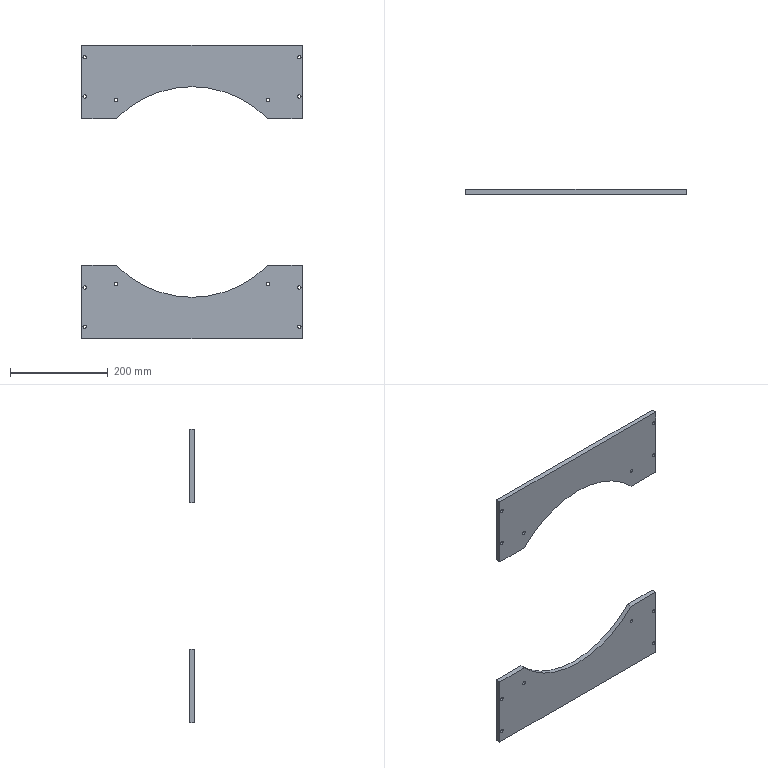Component | SolidWorks | DiscBasePlate-1 | 2 solids | 40 faces | volume 1069204 mm3 | cylinder 26 | plane 14 | commonest cylinder face diameters 7 x16 6.8 x8 430 x2